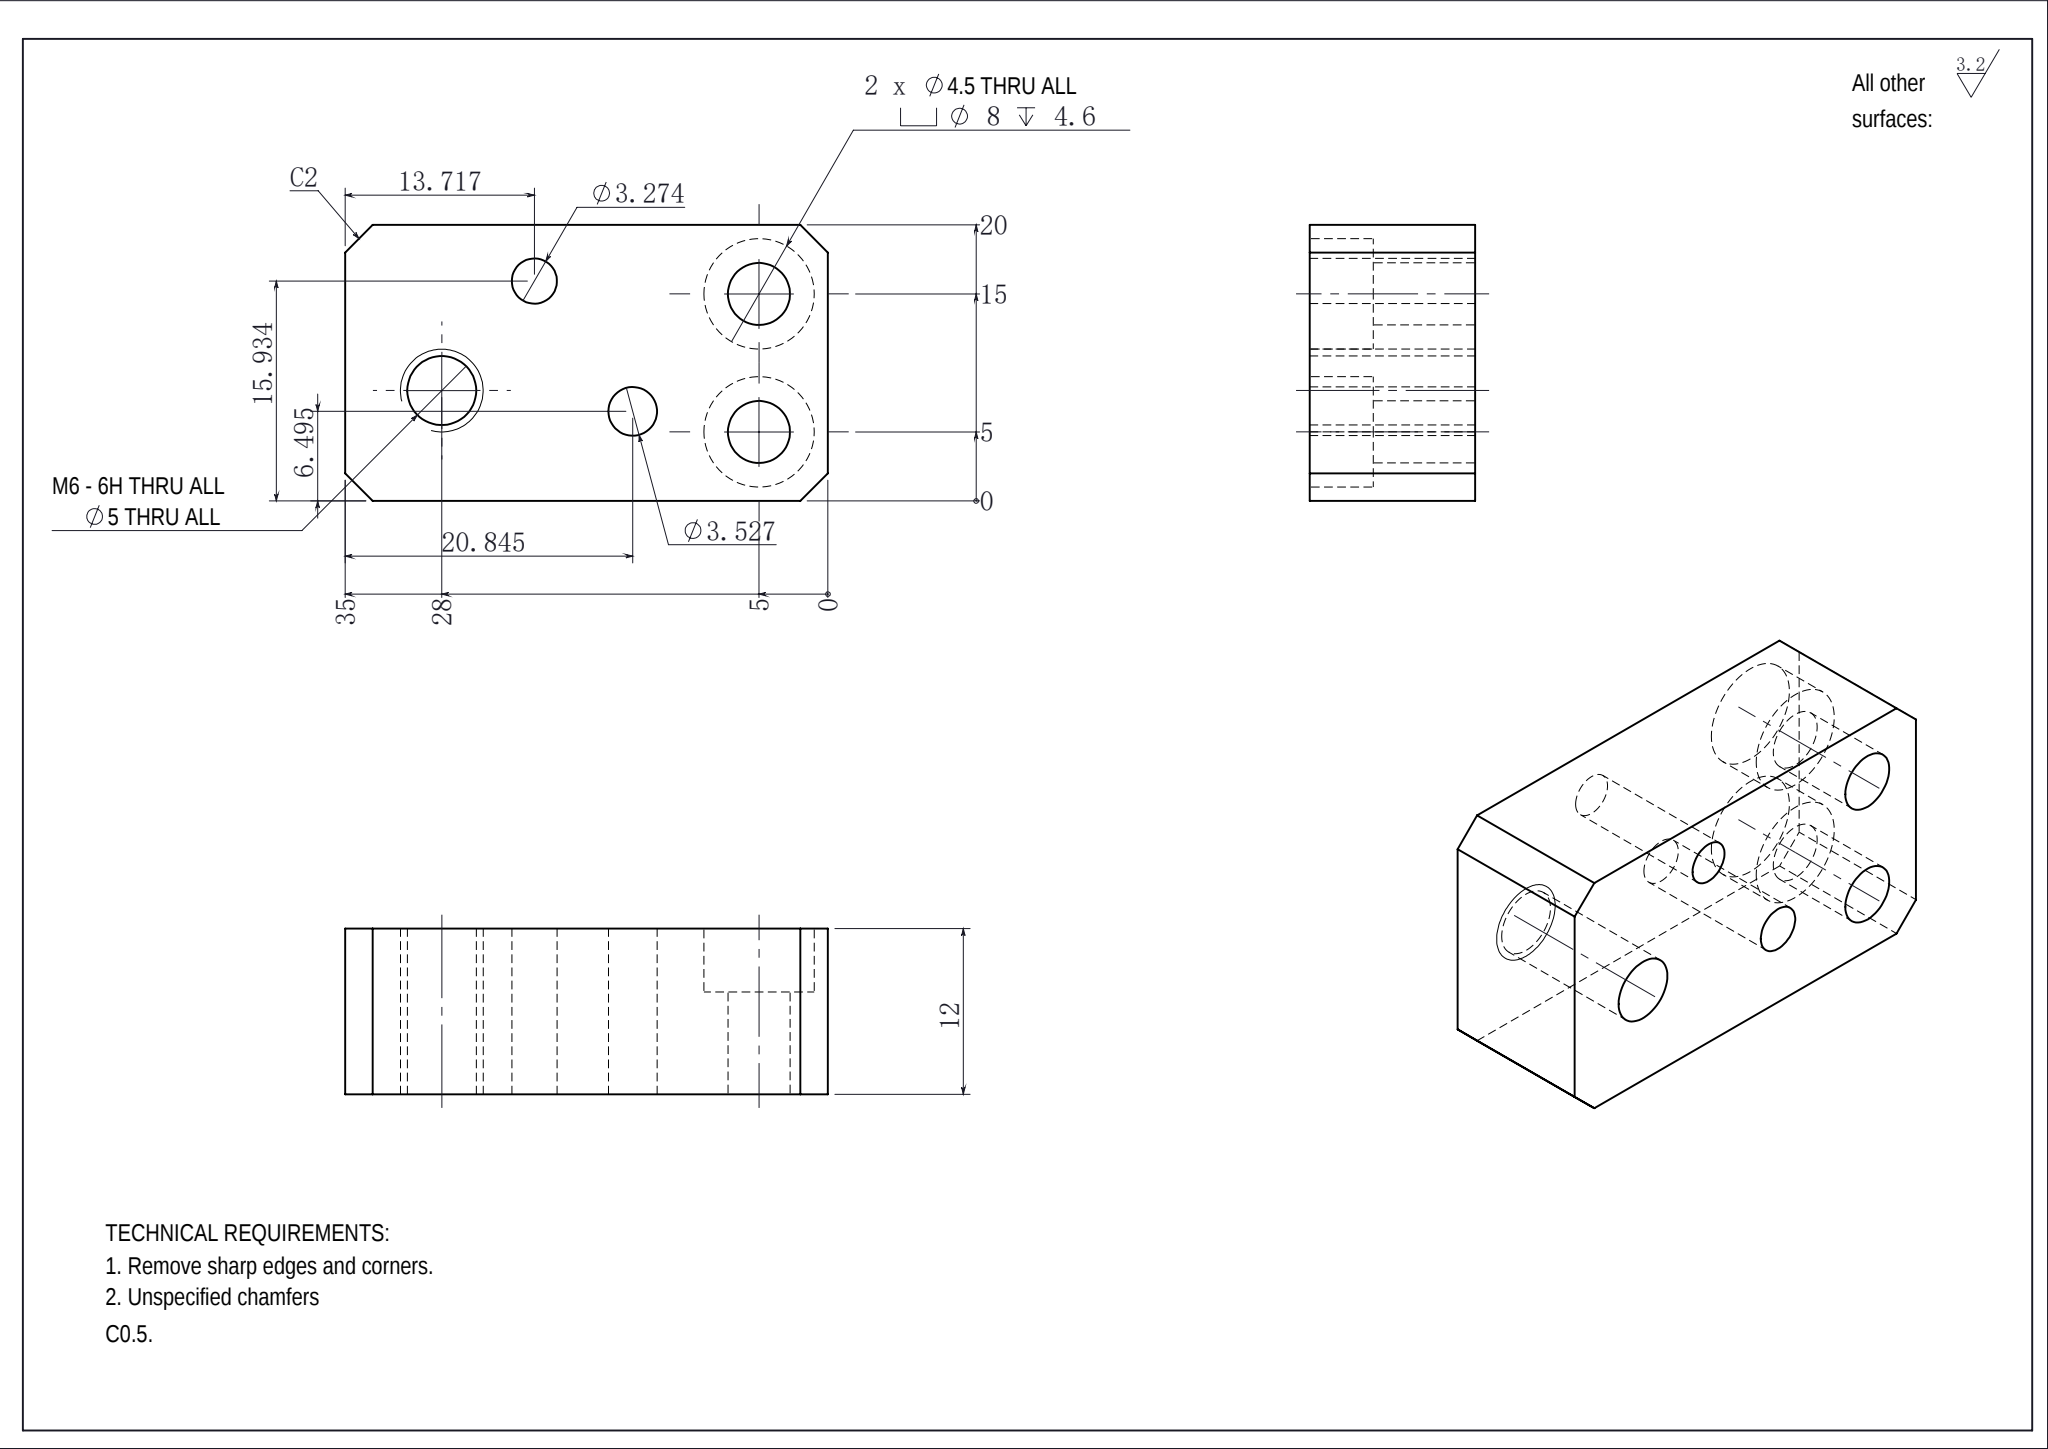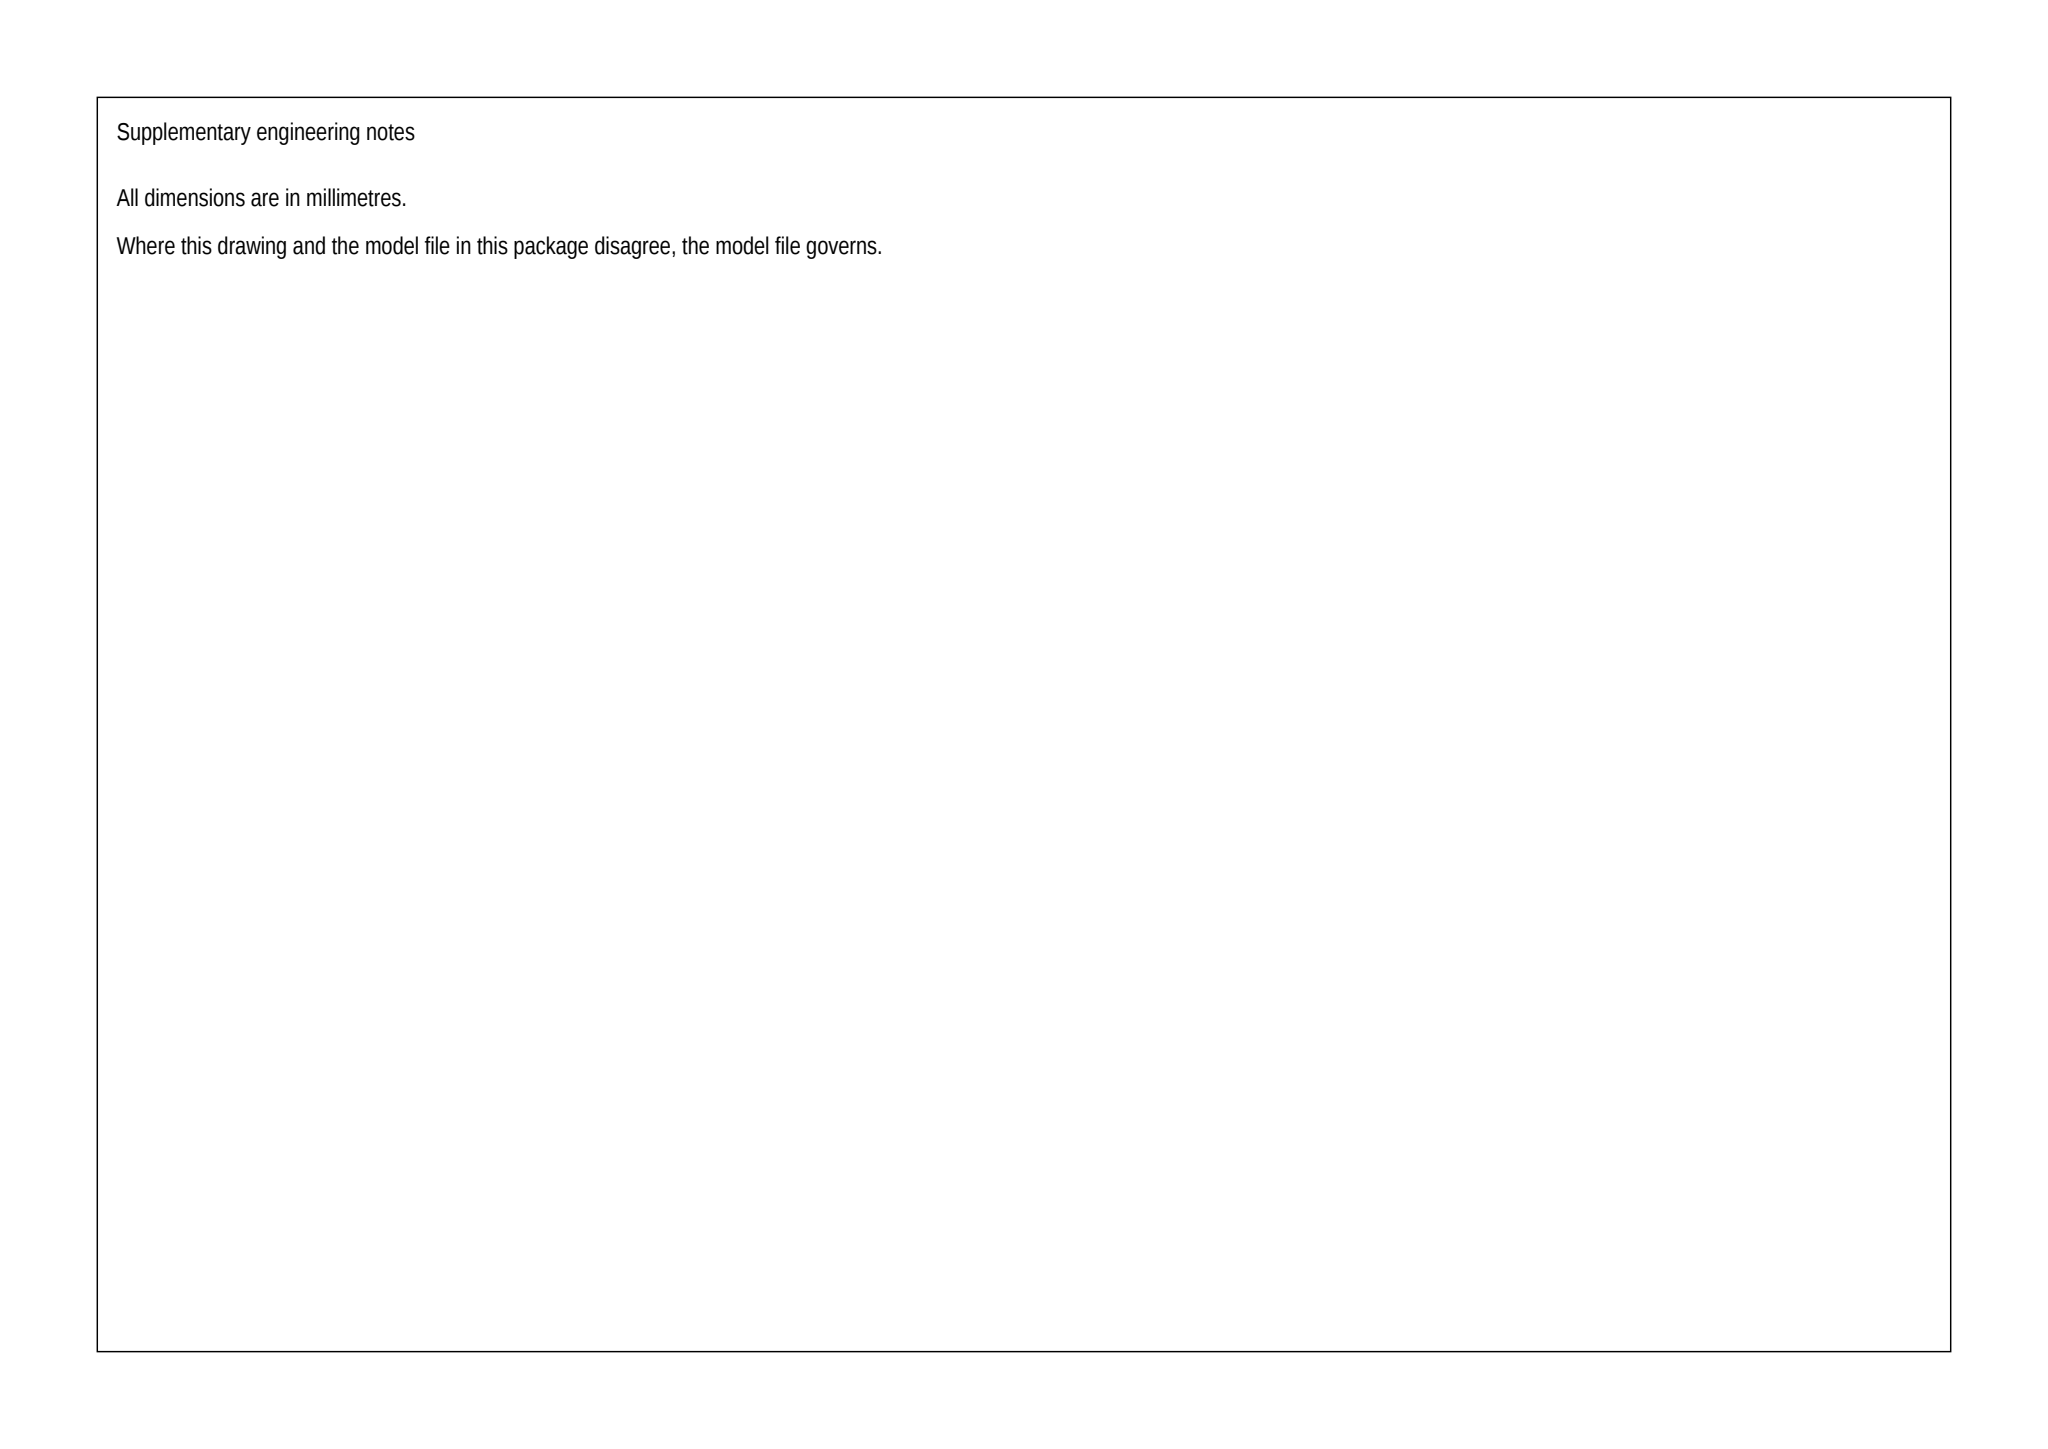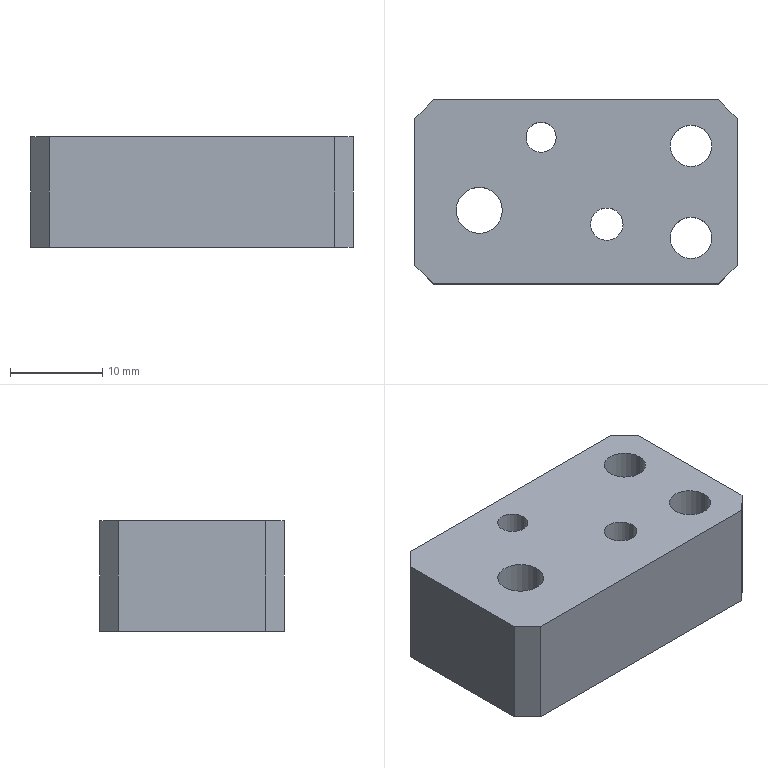Part | SolidWorks | mm | 1 solid | 26 faces | box 35 x 20 x 12 mm | volume 7152 mm3 | cylinder 14 | plane 12 | commonest cylinder face diameters 8 x4 4.5 x4 3.527 x2 3.274 x2 5 x2
build123d program:
from build123d import *

# Parameters (mm, degrees)
SKETCH1_W                                          = 35
SKETCH1_H                                          = 20
BOSS_EXTRUDE1_DEPTH                                = 6
HOLE_SIZE_ACCORDING_TO_TYPE_1_OF_HEXAG_D           = 4.5
HOLE_SIZE_ACCORDING_TO_TYPE_1_OF_HEXAG_CBORE_D     = 8
HOLE_SIZE_ACCORDING_TO_TYPE_1_OF_HEXAG_CBORE_DEPTH = 4.6
M6_TAPPED_HOLE1_D                                  = 5
CHAMFER1_SIZE                                      = 2
SKETCH8_R                                          = 1.764
SKETCH8_R_2                                        = 1.637
CUT_EXTRUDE1_DEPTH                                 = 80


with BuildPart() as part:
    # Sketch1 → Boss-Extrude1 (new, symmetric)
    with BuildSketch(Plane.XY):
        Rectangle(SKETCH1_W, SKETCH1_H)
    extrude(amount=BOSS_EXTRUDE1_DEPTH, both=True)

    # Hole Size _according to_ Type 1 of Hexag (through all)
    with Locations(Plane(origin=(0, 0, -6), x_dir=(-1, 0, 0), z_dir=(0, 0, -1))):
        with Locations((-12.5, 5), (-12.5, -5)):
            CounterBoreHole(HOLE_SIZE_ACCORDING_TO_TYPE_1_OF_HEXAG_D / 2, HOLE_SIZE_ACCORDING_TO_TYPE_1_OF_HEXAG_CBORE_D / 2, HOLE_SIZE_ACCORDING_TO_TYPE_1_OF_HEXAG_CBORE_DEPTH)

    # M6 Tapped Hole1 (through all)
    with Locations(Plane(origin=(0, 0, -6), x_dir=(-1, 0, 0), z_dir=(0, 0, -1))):
        with Locations((10.5, -2)):
            Hole(M6_TAPPED_HOLE1_D / 2)

    # Chamfer1
    chamfer1_edges = [part.edges().sort_by_distance(p)[0] for p in [
        (17.5, -10, 0),
        (-17.5, -10, 0),
        (-17.5, 10, 0),
        (17.5, 10, 0),
    ]]
    chamfer(chamfer1_edges, length=CHAMFER1_SIZE)

    # Sketch8 → Cut-Extrude1 (cut)
    with BuildSketch(Plane(origin=(0, 0, -6), x_dir=(-1, 0, 0), z_dir=(0, 0, -1))):
        with Locations((-3.345, -3.505)):
            Circle(SKETCH8_R)
        with Locations((3.783, 5.934)):
            Circle(SKETCH8_R_2)
    extrude(amount=-CUT_EXTRUDE1_DEPTH, mode=Mode.SUBTRACT)


solid = part.part
STEP:
#1=CARTESIAN_POINT('',(5.109,-3.505,6.));
#2=VERTEX_POINT('',#1);
#3=CARTESIAN_POINT('',(1.582,-3.505,6.));
#4=VERTEX_POINT('',#3);
#5=CARTESIAN_POINT('',(3.345,-3.505,6.));
#6=DIRECTION('',(0.,0.,-1.));
#7=DIRECTION('',(-1.,0.,0.));
#8=AXIS2_PLACEMENT_3D('',#5,#6,#7);
#9=CIRCLE('',#8,1.764);
#10=EDGE_CURVE('',#2,#4,#9,.T.);
#11=ORIENTED_EDGE('',*,*,#10,.F.);
#12=CARTESIAN_POINT('',(5.109,-3.505,-6.));
#13=VERTEX_POINT('',#12);
#14=CARTESIAN_POINT('',(5.109,-3.505,74.));
#15=DIRECTION('',(0.,0.,-1.));
#16=VECTOR('',#15,1000.);
#17=LINE('',#14,#16);
#18=EDGE_CURVE('',#2,#13,#17,.T.);
#19=ORIENTED_EDGE('',*,*,#18,.T.);
#20=CARTESIAN_POINT('',(1.582,-3.505,-6.));
#21=VERTEX_POINT('',#20);
#22=CARTESIAN_POINT('',(3.345,-3.505,-6.));
#23=DIRECTION('',(0.,0.,-1.));
#24=DIRECTION('',(-1.,0.,0.));
#25=AXIS2_PLACEMENT_3D('',#22,#23,#24);
#26=CIRCLE('',#25,1.764);
#27=EDGE_CURVE('',#13,#21,#26,.T.);
#28=ORIENTED_EDGE('',*,*,#27,.T.);
#29=CARTESIAN_POINT('',(1.582,-3.505,74.));
#30=DIRECTION('',(0.,0.,-1.));
#31=VECTOR('',#30,1000.);
#32=LINE('',#29,#31);
#33=EDGE_CURVE('',#4,#21,#32,.T.);
#34=ORIENTED_EDGE('',*,*,#33,.F.);
#35=EDGE_LOOP('',(#11,#19,#28,#34));
#36=FACE_OUTER_BOUND('',#35,.T.);
#37=CARTESIAN_POINT('',(3.345,-3.505,74.));
#38=DIRECTION('',(0.,0.,-1.));
#39=DIRECTION('',(-1.,0.,0.));
#40=AXIS2_PLACEMENT_3D('',#37,#38,#39);
#41=CYLINDRICAL_SURFACE('',#40,1.764);
#42=ADVANCED_FACE('',(#36),#41,.F.);
#43=CARTESIAN_POINT('',(-2.146,5.934,6.));
#44=VERTEX_POINT('',#43);
#45=CARTESIAN_POINT('',(-5.421,5.934,6.));
#46=VERTEX_POINT('',#45);
#47=CARTESIAN_POINT('',(-3.783,5.934,6.));
#48=DIRECTION('',(0.,0.,-1.));
#49=DIRECTION('',(-1.,0.,0.));
#50=AXIS2_PLACEMENT_3D('',#47,#48,#49);
#51=CIRCLE('',#50,1.637);
#52=EDGE_CURVE('',#44,#46,#51,.T.);
#53=ORIENTED_EDGE('',*,*,#52,.F.);
#54=CARTESIAN_POINT('',(-2.146,5.934,-6.));
#55=VERTEX_POINT('',#54);
#56=CARTESIAN_POINT('',(-2.146,5.934,74.));
#57=DIRECTION('',(0.,0.,-1.));
#58=VECTOR('',#57,1000.);
#59=LINE('',#56,#58);
#60=EDGE_CURVE('',#44,#55,#59,.T.);
#61=ORIENTED_EDGE('',*,*,#60,.T.);
#62=CARTESIAN_POINT('',(-5.421,5.934,-6.));
#63=VERTEX_POINT('',#62);
#64=CARTESIAN_POINT('',(-3.783,5.934,-6.));
#65=DIRECTION('',(0.,0.,-1.));
#66=DIRECTION('',(-1.,0.,0.));
#67=AXIS2_PLACEMENT_3D('',#64,#65,#66);
#68=CIRCLE('',#67,1.637);
#69=EDGE_CURVE('',#55,#63,#68,.T.);
#70=ORIENTED_EDGE('',*,*,#69,.T.);
#71=CARTESIAN_POINT('',(-5.421,5.934,74.));
#72=DIRECTION('',(0.,0.,-1.));
#73=VECTOR('',#72,1000.);
#74=LINE('',#71,#73);
#75=EDGE_CURVE('',#46,#63,#74,.T.);
#76=ORIENTED_EDGE('',*,*,#75,.F.);
#77=EDGE_LOOP('',(#53,#61,#70,#76));
#78=FACE_OUTER_BOUND('',#77,.T.);
#79=CARTESIAN_POINT('',(-3.783,5.934,74.));
#80=DIRECTION('',(0.,0.,-1.));
#81=DIRECTION('',(-1.,0.,0.));
#82=AXIS2_PLACEMENT_3D('',#79,#80,#81);
#83=CYLINDRICAL_SURFACE('',#82,1.637);
#84=ADVANCED_FACE('',(#78),#83,.F.);
#85=CARTESIAN_POINT('',(-8.,-2.,6.));
#86=VERTEX_POINT('',#85);
#87=CARTESIAN_POINT('',(-13.,-2.,6.));
#88=VERTEX_POINT('',#87);
#89=CARTESIAN_POINT('',(-10.5,-2.,6.));
#90=DIRECTION('',(0.,0.,-1.));
#91=DIRECTION('',(-1.,0.,0.));
#92=AXIS2_PLACEMENT_3D('',#89,#90,#91);
#93=CIRCLE('',#92,2.5);
#94=EDGE_CURVE('',#86,#88,#93,.T.);
#95=ORIENTED_EDGE('',*,*,#94,.F.);
#96=CARTESIAN_POINT('',(-8.,-2.,-6.));
#97=VERTEX_POINT('',#96);
#98=CARTESIAN_POINT('',(-8.,-2.,-6.));
#99=DIRECTION('',(0.,0.,-1.));
#100=VECTOR('',#99,1000.);
#101=LINE('',#98,#100);
#102=EDGE_CURVE('',#86,#97,#101,.T.);
#103=ORIENTED_EDGE('',*,*,#102,.T.);
#104=CARTESIAN_POINT('',(-13.,-2.,-6.));
#105=VERTEX_POINT('',#104);
#106=CARTESIAN_POINT('',(-10.5,-2.,-6.));
#107=DIRECTION('',(0.,0.,-1.));
#108=DIRECTION('',(-1.,0.,0.));
#109=AXIS2_PLACEMENT_3D('',#106,#107,#108);
#110=CIRCLE('',#109,2.5);
#111=EDGE_CURVE('',#97,#105,#110,.T.);
#112=ORIENTED_EDGE('',*,*,#111,.T.);
#113=CARTESIAN_POINT('',(-13.,-2.,-6.));
#114=DIRECTION('',(0.,0.,-1.));
#115=VECTOR('',#114,1000.);
#116=LINE('',#113,#115);
#117=EDGE_CURVE('',#88,#105,#116,.T.);
#118=ORIENTED_EDGE('',*,*,#117,.F.);
#119=EDGE_LOOP('',(#95,#103,#112,#118));
#120=FACE_OUTER_BOUND('',#119,.T.);
#121=CARTESIAN_POINT('',(-10.5,-2.,-6.));
#122=DIRECTION('',(0.,0.,-1.));
#123=DIRECTION('',(-1.,0.,0.));
#124=AXIS2_PLACEMENT_3D('',#121,#122,#123);
#125=CYLINDRICAL_SURFACE('',#124,2.5);
#126=ADVANCED_FACE('',(#120),#125,.F.);
#127=CARTESIAN_POINT('',(16.5,5.,-1.4));
#128=VERTEX_POINT('',#127);
#129=CARTESIAN_POINT('',(8.5,5.,-1.4));
#130=VERTEX_POINT('',#129);
#131=CARTESIAN_POINT('',(12.5,5.,-1.4));
#132=DIRECTION('',(0.,0.,-1.));
#133=DIRECTION('',(-1.,0.,0.));
#134=AXIS2_PLACEMENT_3D('',#131,#132,#133);
#135=CIRCLE('',#134,4.);
#136=EDGE_CURVE('',#128,#130,#135,.T.);
#137=ORIENTED_EDGE('',*,*,#136,.F.);
#138=CARTESIAN_POINT('',(16.5,5.,-6.));
#139=VERTEX_POINT('',#138);
#140=CARTESIAN_POINT('',(16.5,5.,-6.));
#141=DIRECTION('',(0.,0.,-1.));
#142=VECTOR('',#141,1000.);
#143=LINE('',#140,#142);
#144=EDGE_CURVE('',#128,#139,#143,.T.);
#145=ORIENTED_EDGE('',*,*,#144,.T.);
#146=CARTESIAN_POINT('',(8.5,5.,-6.));
#147=VERTEX_POINT('',#146);
#148=CARTESIAN_POINT('',(12.5,5.,-6.));
#149=DIRECTION('',(0.,0.,-1.));
#150=DIRECTION('',(-1.,0.,0.));
#151=AXIS2_PLACEMENT_3D('',#148,#149,#150);
#152=CIRCLE('',#151,4.);
#153=EDGE_CURVE('',#139,#147,#152,.T.);
#154=ORIENTED_EDGE('',*,*,#153,.T.);
#155=CARTESIAN_POINT('',(8.5,5.,-6.));
#156=DIRECTION('',(0.,0.,-1.));
#157=VECTOR('',#156,1000.);
#158=LINE('',#155,#157);
#159=EDGE_CURVE('',#130,#147,#158,.T.);
#160=ORIENTED_EDGE('',*,*,#159,.F.);
#161=EDGE_LOOP('',(#137,#145,#154,#160));
#162=FACE_OUTER_BOUND('',#161,.T.);
#163=CARTESIAN_POINT('',(12.5,5.,-6.));
#164=DIRECTION('',(0.,0.,-1.));
#165=DIRECTION('',(-1.,0.,0.));
#166=AXIS2_PLACEMENT_3D('',#163,#164,#165);
#167=CYLINDRICAL_SURFACE('',#166,4.);
#168=ADVANCED_FACE('',(#162),#167,.F.);
#169=CARTESIAN_POINT('',(14.75,5.,6.));
#170=VERTEX_POINT('',#169);
#171=CARTESIAN_POINT('',(10.25,5.,6.));
#172=VERTEX_POINT('',#171);
#173=CARTESIAN_POINT('',(12.5,5.,6.));
#174=DIRECTION('',(0.,0.,-1.));
#175=DIRECTION('',(-1.,0.,0.));
#176=AXIS2_PLACEMENT_3D('',#173,#174,#175);
#177=CIRCLE('',#176,2.25);
#178=EDGE_CURVE('',#170,#172,#177,.T.);
#179=ORIENTED_EDGE('',*,*,#178,.F.);
#180=CARTESIAN_POINT('',(14.75,5.,-1.4));
#181=VERTEX_POINT('',#180);
#182=CARTESIAN_POINT('',(14.75,5.,-6.));
#183=DIRECTION('',(0.,0.,-1.));
#184=VECTOR('',#183,1000.);
#185=LINE('',#182,#184);
#186=EDGE_CURVE('',#170,#181,#185,.T.);
#187=ORIENTED_EDGE('',*,*,#186,.T.);
#188=CARTESIAN_POINT('',(10.25,5.,-1.4));
#189=VERTEX_POINT('',#188);
#190=CARTESIAN_POINT('',(12.5,5.,-1.4));
#191=DIRECTION('',(0.,0.,-1.));
#192=DIRECTION('',(-1.,0.,0.));
#193=AXIS2_PLACEMENT_3D('',#190,#191,#192);
#194=CIRCLE('',#193,2.25);
#195=EDGE_CURVE('',#181,#189,#194,.T.);
#196=ORIENTED_EDGE('',*,*,#195,.T.);
#197=CARTESIAN_POINT('',(10.25,5.,-6.));
#198=DIRECTION('',(0.,0.,-1.));
#199=VECTOR('',#198,1000.);
#200=LINE('',#197,#199);
#201=EDGE_CURVE('',#172,#189,#200,.T.);
#202=ORIENTED_EDGE('',*,*,#201,.F.);
#203=EDGE_LOOP('',(#179,#187,#196,#202));
#204=FACE_OUTER_BOUND('',#203,.T.);
#205=CARTESIAN_POINT('',(12.5,5.,-6.));
#206=DIRECTION('',(0.,0.,-1.));
#207=DIRECTION('',(-1.,0.,0.));
#208=AXIS2_PLACEMENT_3D('',#205,#206,#207);
#209=CYLINDRICAL_SURFACE('',#208,2.25);
#210=ADVANCED_FACE('',(#204),#209,.F.);
#211=CARTESIAN_POINT('',(16.5,-5.,-1.4));
#212=VERTEX_POINT('',#211);
#213=CARTESIAN_POINT('',(8.5,-5.,-1.4));
#214=VERTEX_POINT('',#213);
#215=CARTESIAN_POINT('',(12.5,-5.,-1.4));
#216=DIRECTION('',(0.,0.,-1.));
#217=DIRECTION('',(-1.,0.,0.));
#218=AXIS2_PLACEMENT_3D('',#215,#216,#217);
#219=CIRCLE('',#218,4.);
#220=EDGE_CURVE('',#212,#214,#219,.T.);
#221=ORIENTED_EDGE('',*,*,#220,.F.);
#222=CARTESIAN_POINT('',(16.5,-5.,-6.));
#223=VERTEX_POINT('',#222);
#224=CARTESIAN_POINT('',(16.5,-5.,-6.));
#225=DIRECTION('',(0.,0.,-1.));
#226=VECTOR('',#225,1000.);
#227=LINE('',#224,#226);
#228=EDGE_CURVE('',#212,#223,#227,.T.);
#229=ORIENTED_EDGE('',*,*,#228,.T.);
#230=CARTESIAN_POINT('',(8.5,-5.,-6.));
#231=VERTEX_POINT('',#230);
#232=CARTESIAN_POINT('',(12.5,-5.,-6.));
#233=DIRECTION('',(0.,0.,-1.));
#234=DIRECTION('',(-1.,0.,0.));
#235=AXIS2_PLACEMENT_3D('',#232,#233,#234);
#236=CIRCLE('',#235,4.);
#237=EDGE_CURVE('',#223,#231,#236,.T.);
#238=ORIENTED_EDGE('',*,*,#237,.T.);
#239=CARTESIAN_POINT('',(8.5,-5.,-6.));
#240=DIRECTION('',(0.,0.,-1.));
#241=VECTOR('',#240,1000.);
#242=LINE('',#239,#241);
#243=EDGE_CURVE('',#214,#231,#242,.T.);
#244=ORIENTED_EDGE('',*,*,#243,.F.);
#245=EDGE_LOOP('',(#221,#229,#238,#244));
#246=FACE_OUTER_BOUND('',#245,.T.);
#247=CARTESIAN_POINT('',(12.5,-5.,-6.));
#248=DIRECTION('',(0.,0.,-1.));
#249=DIRECTION('',(-1.,0.,0.));
#250=AXIS2_PLACEMENT_3D('',#247,#248,#249);
#251=CYLINDRICAL_SURFACE('',#250,4.);
#252=ADVANCED_FACE('',(#246),#251,.F.);
#253=CARTESIAN_POINT('',(14.75,-5.,6.));
#254=VERTEX_POINT('',#253);
#255=CARTESIAN_POINT('',(10.25,-5.,6.));
#256=VERTEX_POINT('',#255);
#257=CARTESIAN_POINT('',(12.5,-5.,6.));
#258=DIRECTION('',(0.,0.,-1.));
#259=DIRECTION('',(-1.,0.,0.));
#260=AXIS2_PLACEMENT_3D('',#257,#258,#259);
#261=CIRCLE('',#260,2.25);
#262=EDGE_CURVE('',#254,#256,#261,.T.);
#263=ORIENTED_EDGE('',*,*,#262,.F.);
#264=CARTESIAN_POINT('',(14.75,-5.,-1.4));
#265=VERTEX_POINT('',#264);
#266=CARTESIAN_POINT('',(14.75,-5.,-6.));
#267=DIRECTION('',(0.,0.,-1.));
#268=VECTOR('',#267,1000.);
#269=LINE('',#266,#268);
#270=EDGE_CURVE('',#254,#265,#269,.T.);
#271=ORIENTED_EDGE('',*,*,#270,.T.);
#272=CARTESIAN_POINT('',(10.25,-5.,-1.4));
#273=VERTEX_POINT('',#272);
#274=CARTESIAN_POINT('',(12.5,-5.,-1.4));
#275=DIRECTION('',(0.,0.,-1.));
#276=DIRECTION('',(-1.,0.,0.));
#277=AXIS2_PLACEMENT_3D('',#274,#275,#276);
#278=CIRCLE('',#277,2.25);
#279=EDGE_CURVE('',#265,#273,#278,.T.);
#280=ORIENTED_EDGE('',*,*,#279,.T.);
#281=CARTESIAN_POINT('',(10.25,-5.,-6.));
#282=DIRECTION('',(0.,0.,-1.));
#283=VECTOR('',#282,1000.);
#284=LINE('',#281,#283);
#285=EDGE_CURVE('',#256,#273,#284,.T.);
#286=ORIENTED_EDGE('',*,*,#285,.F.);
#287=EDGE_LOOP('',(#263,#271,#280,#286));
#288=FACE_OUTER_BOUND('',#287,.T.);
#289=CARTESIAN_POINT('',(12.5,-5.,-6.));
#290=DIRECTION('',(0.,0.,-1.));
#291=DIRECTION('',(-1.,0.,0.));
#292=AXIS2_PLACEMENT_3D('',#289,#290,#291);
#293=CYLINDRICAL_SURFACE('',#292,2.25);
#294=ADVANCED_FACE('',(#288),#293,.F.);
#295=CARTESIAN_POINT('',(17.5,-8.,6.));
#296=VERTEX_POINT('',#295);
#297=CARTESIAN_POINT('',(17.5,8.,6.));
#298=VERTEX_POINT('',#297);
#299=CARTESIAN_POINT('',(17.5,-10.,6.));
#300=DIRECTION('',(0.,1.,0.));
#301=VECTOR('',#300,1000.);
#302=LINE('',#299,#301);
#303=EDGE_CURVE('',#296,#298,#302,.T.);
#304=ORIENTED_EDGE('',*,*,#303,.F.);
#305=CARTESIAN_POINT('',(17.5,-8.,-6.));
#306=VERTEX_POINT('',#305);
#307=CARTESIAN_POINT('',(17.5,-8.,6.));
#308=DIRECTION('',(0.,0.,-1.));
#309=VECTOR('',#308,1000.);
#310=LINE('',#307,#309);
#311=EDGE_CURVE('',#296,#306,#310,.T.);
#312=ORIENTED_EDGE('',*,*,#311,.T.);
#313=CARTESIAN_POINT('',(17.5,8.,-6.));
#314=VERTEX_POINT('',#313);
#315=CARTESIAN_POINT('',(17.5,-10.,-6.));
#316=DIRECTION('',(0.,1.,0.));
#317=VECTOR('',#316,1000.);
#318=LINE('',#315,#317);
#319=EDGE_CURVE('',#306,#314,#318,.T.);
#320=ORIENTED_EDGE('',*,*,#319,.T.);
#321=CARTESIAN_POINT('',(17.5,8.,6.));
#322=DIRECTION('',(0.,0.,1.));
#323=VECTOR('',#322,1000.);
#324=LINE('',#321,#323);
#325=EDGE_CURVE('',#314,#298,#324,.T.);
#326=ORIENTED_EDGE('',*,*,#325,.T.);
#327=EDGE_LOOP('',(#304,#312,#320,#326));
#328=FACE_OUTER_BOUND('',#327,.T.);
#329=CARTESIAN_POINT('',(17.5,-10.,6.));
#330=DIRECTION('',(-1.,0.,0.));
#331=DIRECTION('',(0.,0.,1.));
#332=AXIS2_PLACEMENT_3D('',#329,#330,#331);
#333=PLANE('',#332);
#334=ADVANCED_FACE('',(#328),#333,.F.);
#335=CARTESIAN_POINT('',(15.5,10.,6.));
#336=VERTEX_POINT('',#335);
#337=CARTESIAN_POINT('',(-15.5,10.,6.));
#338=VERTEX_POINT('',#337);
#339=CARTESIAN_POINT('',(-17.5,10.,6.));
#340=DIRECTION('',(-1.,0.,0.));
#341=VECTOR('',#340,1000.);
#342=LINE('',#339,#341);
#343=EDGE_CURVE('',#336,#338,#342,.T.);
#344=ORIENTED_EDGE('',*,*,#343,.F.);
#345=CARTESIAN_POINT('',(15.5,10.,-6.));
#346=VERTEX_POINT('',#345);
#347=CARTESIAN_POINT('',(15.5,10.,6.));
#348=DIRECTION('',(0.,0.,-1.));
#349=VECTOR('',#348,1000.);
#350=LINE('',#347,#349);
#351=EDGE_CURVE('',#336,#346,#350,.T.);
#352=ORIENTED_EDGE('',*,*,#351,.T.);
#353=CARTESIAN_POINT('',(-15.5,10.,-6.));
#354=VERTEX_POINT('',#353);
#355=CARTESIAN_POINT('',(-17.5,10.,-6.));
#356=DIRECTION('',(-1.,0.,0.));
#357=VECTOR('',#356,1000.);
#358=LINE('',#355,#357);
#359=EDGE_CURVE('',#346,#354,#358,.T.);
#360=ORIENTED_EDGE('',*,*,#359,.T.);
#361=CARTESIAN_POINT('',(-15.5,10.,6.));
#362=DIRECTION('',(0.,0.,1.));
#363=VECTOR('',#362,1000.);
#364=LINE('',#361,#363);
#365=EDGE_CURVE('',#354,#338,#364,.T.);
#366=ORIENTED_EDGE('',*,*,#365,.T.);
#367=EDGE_LOOP('',(#344,#352,#360,#366));
#368=FACE_OUTER_BOUND('',#367,.T.);
#369=CARTESIAN_POINT('',(-17.5,10.,6.));
#370=DIRECTION('',(0.,-1.,0.));
#371=DIRECTION('',(0.,0.,-1.));
#372=AXIS2_PLACEMENT_3D('',#369,#370,#371);
#373=PLANE('',#372);
#374=ADVANCED_FACE('',(#368),#373,.F.);
#375=CARTESIAN_POINT('',(-17.5,8.,-6.));
#376=VERTEX_POINT('',#375);
#377=CARTESIAN_POINT('',(-17.5,-8.,-6.));
#378=VERTEX_POINT('',#377);
#379=CARTESIAN_POINT('',(-17.5,-10.,-6.));
#380=DIRECTION('',(0.,-1.,0.));
#381=VECTOR('',#380,1000.);
#382=LINE('',#379,#381);
#383=EDGE_CURVE('',#376,#378,#382,.T.);
#384=ORIENTED_EDGE('',*,*,#383,.T.);
#385=CARTESIAN_POINT('',(-17.5,-8.,6.));
#386=VERTEX_POINT('',#385);
#387=CARTESIAN_POINT('',(-17.5,-8.,6.));
#388=DIRECTION('',(0.,0.,1.));
#389=VECTOR('',#388,1000.);
#390=LINE('',#387,#389);
#391=EDGE_CURVE('',#378,#386,#390,.T.);
#392=ORIENTED_EDGE('',*,*,#391,.T.);
#393=CARTESIAN_POINT('',(-17.5,8.,6.));
#394=VERTEX_POINT('',#393);
#395=CARTESIAN_POINT('',(-17.5,-10.,6.));
#396=DIRECTION('',(0.,-1.,0.));
#397=VECTOR('',#396,1000.);
#398=LINE('',#395,#397);
#399=EDGE_CURVE('',#394,#386,#398,.T.);
#400=ORIENTED_EDGE('',*,*,#399,.F.);
#401=CARTESIAN_POINT('',(-17.5,8.,6.));
#402=DIRECTION('',(0.,0.,-1.));
#403=VECTOR('',#402,1000.);
#404=LINE('',#401,#403);
#405=EDGE_CURVE('',#394,#376,#404,.T.);
#406=ORIENTED_EDGE('',*,*,#405,.T.);
#407=EDGE_LOOP('',(#384,#392,#400,#406));
#408=FACE_OUTER_BOUND('',#407,.T.);
#409=CARTESIAN_POINT('',(-17.5,-10.,6.));
#410=DIRECTION('',(1.,0.,0.));
#411=DIRECTION('',(0.,0.,-1.));
#412=AXIS2_PLACEMENT_3D('',#409,#410,#411);
#413=PLANE('',#412);
#414=ADVANCED_FACE('',(#408),#413,.F.);
#415=CARTESIAN_POINT('',(-15.5,-10.,6.));
#416=VERTEX_POINT('',#415);
#417=CARTESIAN_POINT('',(15.5,-10.,6.));
#418=VERTEX_POINT('',#417);
#419=CARTESIAN_POINT('',(-17.5,-10.,6.));
#420=DIRECTION('',(1.,0.,0.));
#421=VECTOR('',#420,1000.);
#422=LINE('',#419,#421);
#423=EDGE_CURVE('',#416,#418,#422,.T.);
#424=ORIENTED_EDGE('',*,*,#423,.F.);
#425=CARTESIAN_POINT('',(-15.5,-10.,-6.));
#426=VERTEX_POINT('',#425);
#427=CARTESIAN_POINT('',(-15.5,-10.,6.));
#428=DIRECTION('',(0.,0.,-1.));
#429=VECTOR('',#428,1000.);
#430=LINE('',#427,#429);
#431=EDGE_CURVE('',#416,#426,#430,.T.);
#432=ORIENTED_EDGE('',*,*,#431,.T.);
#433=CARTESIAN_POINT('',(15.5,-10.,-6.));
#434=VERTEX_POINT('',#433);
#435=CARTESIAN_POINT('',(-17.5,-10.,-6.));
#436=DIRECTION('',(1.,0.,0.));
#437=VECTOR('',#436,1000.);
#438=LINE('',#435,#437);
#439=EDGE_CURVE('',#426,#434,#438,.T.);
#440=ORIENTED_EDGE('',*,*,#439,.T.);
#441=CARTESIAN_POINT('',(15.5,-10.,6.));
#442=DIRECTION('',(0.,0.,1.));
#443=VECTOR('',#442,1000.);
#444=LINE('',#441,#443);
#445=EDGE_CURVE('',#434,#418,#444,.T.);
#446=ORIENTED_EDGE('',*,*,#445,.T.);
#447=EDGE_LOOP('',(#424,#432,#440,#446));
#448=FACE_OUTER_BOUND('',#447,.T.);
#449=CARTESIAN_POINT('',(-17.5,-10.,6.));
#450=DIRECTION('',(0.,1.,0.));
#451=DIRECTION('',(0.,0.,1.));
#452=AXIS2_PLACEMENT_3D('',#449,#450,#451);
#453=PLANE('',#452);
#454=ADVANCED_FACE('',(#448),#453,.F.);
#455=CARTESIAN_POINT('',(3.345,-3.505,6.));
#456=DIRECTION('',(0.,0.,-1.));
#457=DIRECTION('',(-1.,0.,0.));
#458=AXIS2_PLACEMENT_3D('',#455,#456,#457);
#459=CIRCLE('',#458,1.764);
#460=EDGE_CURVE('',#4,#2,#459,.T.);
#461=ORIENTED_EDGE('',*,*,#460,.T.);
#462=ORIENTED_EDGE('',*,*,#10,.T.);
#463=EDGE_LOOP('',(#461,#462));
#464=FACE_BOUND('',#463,.T.);
#465=CARTESIAN_POINT('',(-3.783,5.934,6.));
#466=DIRECTION('',(0.,0.,-1.));
#467=DIRECTION('',(-1.,0.,0.));
#468=AXIS2_PLACEMENT_3D('',#465,#466,#467);
#469=CIRCLE('',#468,1.637);
#470=EDGE_CURVE('',#46,#44,#469,.T.);
#471=ORIENTED_EDGE('',*,*,#470,.T.);
#472=ORIENTED_EDGE('',*,*,#52,.T.);
#473=EDGE_LOOP('',(#471,#472));
#474=FACE_BOUND('',#473,.T.);
#475=CARTESIAN_POINT('',(-10.5,-2.,6.));
#476=DIRECTION('',(0.,0.,-1.));
#477=DIRECTION('',(-1.,0.,0.));
#478=AXIS2_PLACEMENT_3D('',#475,#476,#477);
#479=CIRCLE('',#478,2.5);
#480=EDGE_CURVE('',#88,#86,#479,.T.);
#481=ORIENTED_EDGE('',*,*,#480,.T.);
#482=ORIENTED_EDGE('',*,*,#94,.T.);
#483=EDGE_LOOP('',(#481,#482));
#484=FACE_BOUND('',#483,.T.);
#485=CARTESIAN_POINT('',(12.5,5.,6.));
#486=DIRECTION('',(0.,0.,-1.));
#487=DIRECTION('',(-1.,0.,0.));
#488=AXIS2_PLACEMENT_3D('',#485,#486,#487);
#489=CIRCLE('',#488,2.25);
#490=EDGE_CURVE('',#172,#170,#489,.T.);
#491=ORIENTED_EDGE('',*,*,#490,.T.);
#492=ORIENTED_EDGE('',*,*,#178,.T.);
#493=EDGE_LOOP('',(#491,#492));
#494=FACE_BOUND('',#493,.T.);
#495=CARTESIAN_POINT('',(12.5,-5.,6.));
#496=DIRECTION('',(0.,0.,-1.));
#497=DIRECTION('',(-1.,0.,0.));
#498=AXIS2_PLACEMENT_3D('',#495,#496,#497);
#499=CIRCLE('',#498,2.25);
#500=EDGE_CURVE('',#256,#254,#499,.T.);
#501=ORIENTED_EDGE('',*,*,#500,.T.);
#502=ORIENTED_EDGE('',*,*,#262,.T.);
#503=EDGE_LOOP('',(#501,#502));
#504=FACE_BOUND('',#503,.T.);
#505=ORIENTED_EDGE('',*,*,#399,.T.);
#506=CARTESIAN_POINT('',(-15.5,-10.,6.));
#507=DIRECTION('',(0.7071,-0.7071,0.));
#508=VECTOR('',#507,1000.);
#509=LINE('',#506,#508);
#510=EDGE_CURVE('',#386,#416,#509,.T.);
#511=ORIENTED_EDGE('',*,*,#510,.T.);
#512=ORIENTED_EDGE('',*,*,#423,.T.);
#513=CARTESIAN_POINT('',(17.5,-8.,6.));
#514=DIRECTION('',(0.7071,0.7071,0.));
#515=VECTOR('',#514,1000.);
#516=LINE('',#513,#515);
#517=EDGE_CURVE('',#418,#296,#516,.T.);
#518=ORIENTED_EDGE('',*,*,#517,.T.);
#519=ORIENTED_EDGE('',*,*,#303,.T.);
#520=CARTESIAN_POINT('',(15.5,10.,6.));
#521=DIRECTION('',(-0.7071,0.7071,0.));
#522=VECTOR('',#521,1000.);
#523=LINE('',#520,#522);
#524=EDGE_CURVE('',#298,#336,#523,.T.);
#525=ORIENTED_EDGE('',*,*,#524,.T.);
#526=ORIENTED_EDGE('',*,*,#343,.T.);
#527=CARTESIAN_POINT('',(-17.5,8.,6.));
#528=DIRECTION('',(-0.7071,-0.7071,0.));
#529=VECTOR('',#528,1000.);
#530=LINE('',#527,#529);
#531=EDGE_CURVE('',#338,#394,#530,.T.);
#532=ORIENTED_EDGE('',*,*,#531,.T.);
#533=EDGE_LOOP('',(#505,#511,#512,#518,#519,#525,#526,#532));
#534=FACE_OUTER_BOUND('',#533,.T.);
#535=CARTESIAN_POINT('',(0.,0.,6.));
#536=DIRECTION('',(0.,0.,-1.));
#537=DIRECTION('',(-1.,0.,0.));
#538=AXIS2_PLACEMENT_3D('',#535,#536,#537);
#539=PLANE('',#538);
#540=ADVANCED_FACE('',(#464,#474,#484,#494,#504,#534),#539,.F.);
#541=CARTESIAN_POINT('',(3.345,-3.505,-6.));
#542=DIRECTION('',(0.,0.,-1.));
#543=DIRECTION('',(-1.,0.,0.));
#544=AXIS2_PLACEMENT_3D('',#541,#542,#543);
#545=CIRCLE('',#544,1.764);
#546=EDGE_CURVE('',#21,#13,#545,.T.);
#547=ORIENTED_EDGE('',*,*,#546,.F.);
#548=ORIENTED_EDGE('',*,*,#27,.F.);
#549=EDGE_LOOP('',(#547,#548));
#550=FACE_BOUND('',#549,.T.);
#551=CARTESIAN_POINT('',(-3.783,5.934,-6.));
#552=DIRECTION('',(0.,0.,-1.));
#553=DIRECTION('',(-1.,0.,0.));
#554=AXIS2_PLACEMENT_3D('',#551,#552,#553);
#555=CIRCLE('',#554,1.637);
#556=EDGE_CURVE('',#63,#55,#555,.T.);
#557=ORIENTED_EDGE('',*,*,#556,.F.);
#558=ORIENTED_EDGE('',*,*,#69,.F.);
#559=EDGE_LOOP('',(#557,#558));
#560=FACE_BOUND('',#559,.T.);
#561=CARTESIAN_POINT('',(-10.5,-2.,-6.));
#562=DIRECTION('',(0.,0.,-1.));
#563=DIRECTION('',(-1.,0.,0.));
#564=AXIS2_PLACEMENT_3D('',#561,#562,#563);
#565=CIRCLE('',#564,2.5);
#566=EDGE_CURVE('',#105,#97,#565,.T.);
#567=ORIENTED_EDGE('',*,*,#566,.F.);
#568=ORIENTED_EDGE('',*,*,#111,.F.);
#569=EDGE_LOOP('',(#567,#568));
#570=FACE_BOUND('',#569,.T.);
#571=CARTESIAN_POINT('',(12.5,5.,-6.));
#572=DIRECTION('',(0.,0.,-1.));
#573=DIRECTION('',(-1.,0.,0.));
#574=AXIS2_PLACEMENT_3D('',#571,#572,#573);
#575=CIRCLE('',#574,4.);
#576=EDGE_CURVE('',#147,#139,#575,.T.);
#577=ORIENTED_EDGE('',*,*,#576,.F.);
#578=ORIENTED_EDGE('',*,*,#153,.F.);
#579=EDGE_LOOP('',(#577,#578));
#580=FACE_BOUND('',#579,.T.);
#581=CARTESIAN_POINT('',(12.5,-5.,-6.));
#582=DIRECTION('',(0.,0.,-1.));
#583=DIRECTION('',(-1.,0.,0.));
#584=AXIS2_PLACEMENT_3D('',#581,#582,#583);
#585=CIRCLE('',#584,4.);
#586=EDGE_CURVE('',#231,#223,#585,.T.);
#587=ORIENTED_EDGE('',*,*,#586,.F.);
#588=ORIENTED_EDGE('',*,*,#237,.F.);
#589=EDGE_LOOP('',(#587,#588));
#590=FACE_BOUND('',#589,.T.);
#591=ORIENTED_EDGE('',*,*,#439,.F.);
#592=CARTESIAN_POINT('',(-12.75,-12.75,-6.));
#593=DIRECTION('',(-0.7071,0.7071,0.));
#594=VECTOR('',#593,1000.);
#595=LINE('',#592,#594);
#596=EDGE_CURVE('',#426,#378,#595,.T.);
#597=ORIENTED_EDGE('',*,*,#596,.T.);
#598=ORIENTED_EDGE('',*,*,#383,.F.);
#599=CARTESIAN_POINT('',(-12.75,12.75,-6.));
#600=DIRECTION('',(0.7071,0.7071,0.));
#601=VECTOR('',#600,1000.);
#602=LINE('',#599,#601);
#603=EDGE_CURVE('',#376,#354,#602,.T.);
#604=ORIENTED_EDGE('',*,*,#603,.T.);
#605=ORIENTED_EDGE('',*,*,#359,.F.);
#606=CARTESIAN_POINT('',(12.75,12.75,-6.));
#607=DIRECTION('',(0.7071,-0.7071,0.));
#608=VECTOR('',#607,1000.);
#609=LINE('',#606,#608);
#610=EDGE_CURVE('',#346,#314,#609,.T.);
#611=ORIENTED_EDGE('',*,*,#610,.T.);
#612=ORIENTED_EDGE('',*,*,#319,.F.);
#613=CARTESIAN_POINT('',(12.75,-12.75,-6.));
#614=DIRECTION('',(-0.7071,-0.7071,0.));
#615=VECTOR('',#614,1000.);
#616=LINE('',#613,#615);
#617=EDGE_CURVE('',#306,#434,#616,.T.);
#618=ORIENTED_EDGE('',*,*,#617,.T.);
#619=EDGE_LOOP('',(#591,#597,#598,#604,#605,#611,#612,#618));
#620=FACE_OUTER_BOUND('',#619,.T.);
#621=CARTESIAN_POINT('',(0.,0.,-6.));
#622=DIRECTION('',(0.,0.,-1.));
#623=DIRECTION('',(-1.,0.,0.));
#624=AXIS2_PLACEMENT_3D('',#621,#622,#623);
#625=PLANE('',#624);
#626=ADVANCED_FACE('',(#550,#560,#570,#580,#590,#620),#625,.T.);
#627=ORIENTED_EDGE('',*,*,#270,.F.);
#628=ORIENTED_EDGE('',*,*,#500,.F.);
#629=ORIENTED_EDGE('',*,*,#285,.T.);
#630=CARTESIAN_POINT('',(12.5,-5.,-1.4));
#631=DIRECTION('',(0.,0.,-1.));
#632=DIRECTION('',(-1.,0.,0.));
#633=AXIS2_PLACEMENT_3D('',#630,#631,#632);
#634=CIRCLE('',#633,2.25);
#635=EDGE_CURVE('',#273,#265,#634,.T.);
#636=ORIENTED_EDGE('',*,*,#635,.T.);
#637=EDGE_LOOP('',(#627,#628,#629,#636));
#638=FACE_OUTER_BOUND('',#637,.T.);
#639=CARTESIAN_POINT('',(12.5,-5.,-6.));
#640=DIRECTION('',(0.,0.,-1.));
#641=DIRECTION('',(-1.,0.,0.));
#642=AXIS2_PLACEMENT_3D('',#639,#640,#641);
#643=CYLINDRICAL_SURFACE('',#642,2.25);
#644=ADVANCED_FACE('',(#638),#643,.F.);
#645=ORIENTED_EDGE('',*,*,#635,.F.);
#646=ORIENTED_EDGE('',*,*,#279,.F.);
#647=EDGE_LOOP('',(#645,#646));
#648=FACE_BOUND('',#647,.T.);
#649=CARTESIAN_POINT('',(12.5,-5.,-1.4));
#650=DIRECTION('',(0.,0.,-1.));
#651=DIRECTION('',(-1.,0.,0.));
#652=AXIS2_PLACEMENT_3D('',#649,#650,#651);
#653=CIRCLE('',#652,4.);
#654=EDGE_CURVE('',#214,#212,#653,.T.);
#655=ORIENTED_EDGE('',*,*,#654,.T.);
#656=ORIENTED_EDGE('',*,*,#220,.T.);
#657=EDGE_LOOP('',(#655,#656));
#658=FACE_OUTER_BOUND('',#657,.T.);
#659=CARTESIAN_POINT('',(14.75,-5.,-1.4));
#660=DIRECTION('',(0.,0.,1.));
#661=DIRECTION('',(1.,0.,0.));
#662=AXIS2_PLACEMENT_3D('',#659,#660,#661);
#663=PLANE('',#662);
#664=ADVANCED_FACE('',(#648,#658),#663,.F.);
#665=ORIENTED_EDGE('',*,*,#228,.F.);
#666=ORIENTED_EDGE('',*,*,#654,.F.);
#667=ORIENTED_EDGE('',*,*,#243,.T.);
#668=ORIENTED_EDGE('',*,*,#586,.T.);
#669=EDGE_LOOP('',(#665,#666,#667,#668));
#670=FACE_OUTER_BOUND('',#669,.T.);
#671=CARTESIAN_POINT('',(12.5,-5.,-6.));
#672=DIRECTION('',(0.,0.,-1.));
#673=DIRECTION('',(-1.,0.,0.));
#674=AXIS2_PLACEMENT_3D('',#671,#672,#673);
#675=CYLINDRICAL_SURFACE('',#674,4.);
#676=ADVANCED_FACE('',(#670),#675,.F.);
#677=ORIENTED_EDGE('',*,*,#186,.F.);
#678=ORIENTED_EDGE('',*,*,#490,.F.);
#679=ORIENTED_EDGE('',*,*,#201,.T.);
#680=CARTESIAN_POINT('',(12.5,5.,-1.4));
#681=DIRECTION('',(0.,0.,-1.));
#682=DIRECTION('',(-1.,0.,0.));
#683=AXIS2_PLACEMENT_3D('',#680,#681,#682);
#684=CIRCLE('',#683,2.25);
#685=EDGE_CURVE('',#189,#181,#684,.T.);
#686=ORIENTED_EDGE('',*,*,#685,.T.);
#687=EDGE_LOOP('',(#677,#678,#679,#686));
#688=FACE_OUTER_BOUND('',#687,.T.);
#689=CARTESIAN_POINT('',(12.5,5.,-6.));
#690=DIRECTION('',(0.,0.,-1.));
#691=DIRECTION('',(-1.,0.,0.));
#692=AXIS2_PLACEMENT_3D('',#689,#690,#691);
#693=CYLINDRICAL_SURFACE('',#692,2.25);
#694=ADVANCED_FACE('',(#688),#693,.F.);
#695=ORIENTED_EDGE('',*,*,#685,.F.);
#696=ORIENTED_EDGE('',*,*,#195,.F.);
#697=EDGE_LOOP('',(#695,#696));
#698=FACE_BOUND('',#697,.T.);
#699=CARTESIAN_POINT('',(12.5,5.,-1.4));
#700=DIRECTION('',(0.,0.,-1.));
#701=DIRECTION('',(-1.,0.,0.));
#702=AXIS2_PLACEMENT_3D('',#699,#700,#701);
#703=CIRCLE('',#702,4.);
#704=EDGE_CURVE('',#130,#128,#703,.T.);
#705=ORIENTED_EDGE('',*,*,#704,.T.);
#706=ORIENTED_EDGE('',*,*,#136,.T.);
#707=EDGE_LOOP('',(#705,#706));
#708=FACE_OUTER_BOUND('',#707,.T.);
#709=CARTESIAN_POINT('',(14.75,5.,-1.4));
#710=DIRECTION('',(0.,0.,1.));
#711=DIRECTION('',(1.,0.,0.));
#712=AXIS2_PLACEMENT_3D('',#709,#710,#711);
#713=PLANE('',#712);
#714=ADVANCED_FACE('',(#698,#708),#713,.F.);
#715=ORIENTED_EDGE('',*,*,#144,.F.);
#716=ORIENTED_EDGE('',*,*,#704,.F.);
#717=ORIENTED_EDGE('',*,*,#159,.T.);
#718=ORIENTED_EDGE('',*,*,#576,.T.);
#719=EDGE_LOOP('',(#715,#716,#717,#718));
#720=FACE_OUTER_BOUND('',#719,.T.);
#721=CARTESIAN_POINT('',(12.5,5.,-6.));
#722=DIRECTION('',(0.,0.,-1.));
#723=DIRECTION('',(-1.,0.,0.));
#724=AXIS2_PLACEMENT_3D('',#721,#722,#723);
#725=CYLINDRICAL_SURFACE('',#724,4.);
#726=ADVANCED_FACE('',(#720),#725,.F.);
#727=ORIENTED_EDGE('',*,*,#102,.F.);
#728=ORIENTED_EDGE('',*,*,#480,.F.);
#729=ORIENTED_EDGE('',*,*,#117,.T.);
#730=ORIENTED_EDGE('',*,*,#566,.T.);
#731=EDGE_LOOP('',(#727,#728,#729,#730));
#732=FACE_OUTER_BOUND('',#731,.T.);
#733=CARTESIAN_POINT('',(-10.5,-2.,-6.));
#734=DIRECTION('',(0.,0.,-1.));
#735=DIRECTION('',(-1.,0.,0.));
#736=AXIS2_PLACEMENT_3D('',#733,#734,#735);
#737=CYLINDRICAL_SURFACE('',#736,2.5);
#738=ADVANCED_FACE('',(#732),#737,.F.);
#739=ORIENTED_EDGE('',*,*,#510,.F.);
#740=ORIENTED_EDGE('',*,*,#391,.F.);
#741=ORIENTED_EDGE('',*,*,#596,.F.);
#742=ORIENTED_EDGE('',*,*,#431,.F.);
#743=EDGE_LOOP('',(#739,#740,#741,#742));
#744=FACE_OUTER_BOUND('',#743,.T.);
#745=CARTESIAN_POINT('',(-15.5,-10.,6.));
#746=DIRECTION('',(0.7071,0.7071,0.));
#747=DIRECTION('',(0.,0.,-1.));
#748=AXIS2_PLACEMENT_3D('',#745,#746,#747);
#749=PLANE('',#748);
#750=ADVANCED_FACE('',(#744),#749,.F.);
#751=ORIENTED_EDGE('',*,*,#517,.F.);
#752=ORIENTED_EDGE('',*,*,#445,.F.);
#753=ORIENTED_EDGE('',*,*,#617,.F.);
#754=ORIENTED_EDGE('',*,*,#311,.F.);
#755=EDGE_LOOP('',(#751,#752,#753,#754));
#756=FACE_OUTER_BOUND('',#755,.T.);
#757=CARTESIAN_POINT('',(17.5,-8.,6.));
#758=DIRECTION('',(-0.7071,0.7071,0.));
#759=DIRECTION('',(0.,0.,-1.));
#760=AXIS2_PLACEMENT_3D('',#757,#758,#759);
#761=PLANE('',#760);
#762=ADVANCED_FACE('',(#756),#761,.F.);
#763=ORIENTED_EDGE('',*,*,#524,.F.);
#764=ORIENTED_EDGE('',*,*,#325,.F.);
#765=ORIENTED_EDGE('',*,*,#610,.F.);
#766=ORIENTED_EDGE('',*,*,#351,.F.);
#767=EDGE_LOOP('',(#763,#764,#765,#766));
#768=FACE_OUTER_BOUND('',#767,.T.);
#769=CARTESIAN_POINT('',(15.5,10.,6.));
#770=DIRECTION('',(-0.7071,-0.7071,0.));
#771=DIRECTION('',(0.,0.,-1.));
#772=AXIS2_PLACEMENT_3D('',#769,#770,#771);
#773=PLANE('',#772);
#774=ADVANCED_FACE('',(#768),#773,.F.);
#775=ORIENTED_EDGE('',*,*,#531,.F.);
#776=ORIENTED_EDGE('',*,*,#365,.F.);
#777=ORIENTED_EDGE('',*,*,#603,.F.);
#778=ORIENTED_EDGE('',*,*,#405,.F.);
#779=EDGE_LOOP('',(#775,#776,#777,#778));
#780=FACE_OUTER_BOUND('',#779,.T.);
#781=CARTESIAN_POINT('',(-17.5,8.,6.));
#782=DIRECTION('',(0.7071,-0.7071,0.));
#783=DIRECTION('',(0.,0.,-1.));
#784=AXIS2_PLACEMENT_3D('',#781,#782,#783);
#785=PLANE('',#784);
#786=ADVANCED_FACE('',(#780),#785,.F.);
#787=ORIENTED_EDGE('',*,*,#60,.F.);
#788=ORIENTED_EDGE('',*,*,#470,.F.);
#789=ORIENTED_EDGE('',*,*,#75,.T.);
#790=ORIENTED_EDGE('',*,*,#556,.T.);
#791=EDGE_LOOP('',(#787,#788,#789,#790));
#792=FACE_OUTER_BOUND('',#791,.T.);
#793=CARTESIAN_POINT('',(-3.783,5.934,74.));
#794=DIRECTION('',(0.,0.,-1.));
#795=DIRECTION('',(-1.,0.,0.));
#796=AXIS2_PLACEMENT_3D('',#793,#794,#795);
#797=CYLINDRICAL_SURFACE('',#796,1.637);
#798=ADVANCED_FACE('',(#792),#797,.F.);
#799=ORIENTED_EDGE('',*,*,#18,.F.);
#800=ORIENTED_EDGE('',*,*,#460,.F.);
#801=ORIENTED_EDGE('',*,*,#33,.T.);
#802=ORIENTED_EDGE('',*,*,#546,.T.);
#803=EDGE_LOOP('',(#799,#800,#801,#802));
#804=FACE_OUTER_BOUND('',#803,.T.);
#805=CARTESIAN_POINT('',(3.345,-3.505,74.));
#806=DIRECTION('',(0.,0.,-1.));
#807=DIRECTION('',(-1.,0.,0.));
#808=AXIS2_PLACEMENT_3D('',#805,#806,#807);
#809=CYLINDRICAL_SURFACE('',#808,1.764);
#810=ADVANCED_FACE('',(#804),#809,.F.);
#811=CLOSED_SHELL('',(#42,#84,#126,#168,#210,#252,#294,#334,#374,#414,#454,#540,#626,#644,#664,#676,#694,#714,#726,#738,#750,#762,#774,#786,#798,#810));
#812=MANIFOLD_SOLID_BREP('',#811);
#813=CARTESIAN_POINT('',(0.,0.,0.));
#814=DIRECTION('',(0.,0.,1.));
#815=DIRECTION('',(1.,0.,0.));
#816=AXIS2_PLACEMENT_3D('',#813,#814,#815);
#817=(LENGTH_UNIT()NAMED_UNIT(*)SI_UNIT(.MILLI.,.METRE.));
#818=UNCERTAINTY_MEASURE_WITH_UNIT(LENGTH_MEASURE(0.00001),#817,'','');
#819=(NAMED_UNIT(*)PLANE_ANGLE_UNIT()SI_UNIT($,.RADIAN.));
#820=(NAMED_UNIT(*)SI_UNIT($,.STERADIAN.)SOLID_ANGLE_UNIT());
#821=(GEOMETRIC_REPRESENTATION_CONTEXT(3)GLOBAL_UNCERTAINTY_ASSIGNED_CONTEXT((#818))GLOBAL_UNIT_ASSIGNED_CONTEXT((#817,#819,#820))REPRESENTATION_CONTEXT('',''));
#822=ADVANCED_BREP_SHAPE_REPRESENTATION('',(#812,#816),#821);